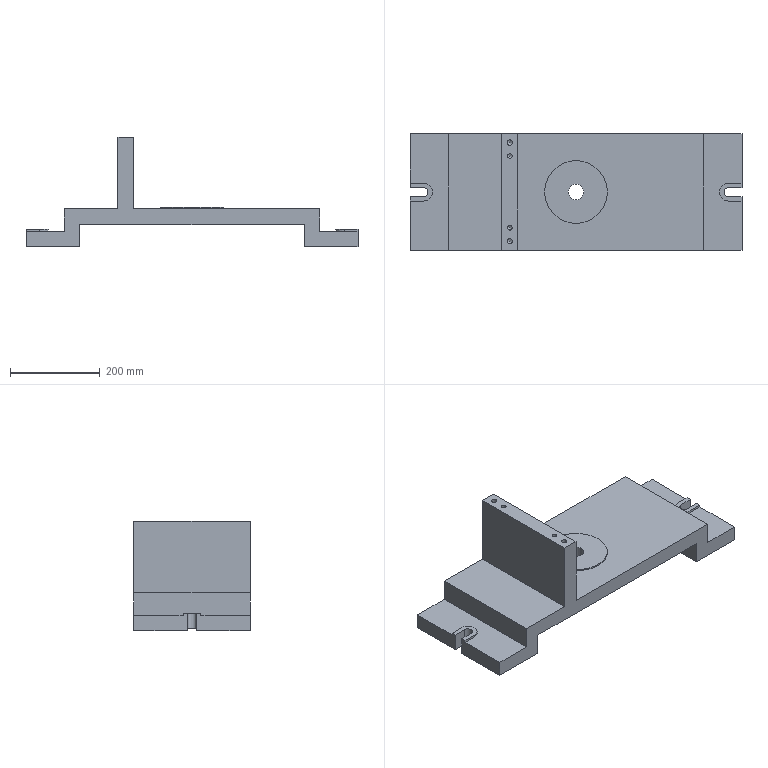Component | NX | FIXTURE_BODY | 1 solid | 53 faces | volume 9038247 mm3 | plane 35 | cylinder 12 | cone 6 | commonest cylinder face diameters 20 x2 40 x2 5.795 x2 11.701 x2 10 x2 140 x1 35 x1